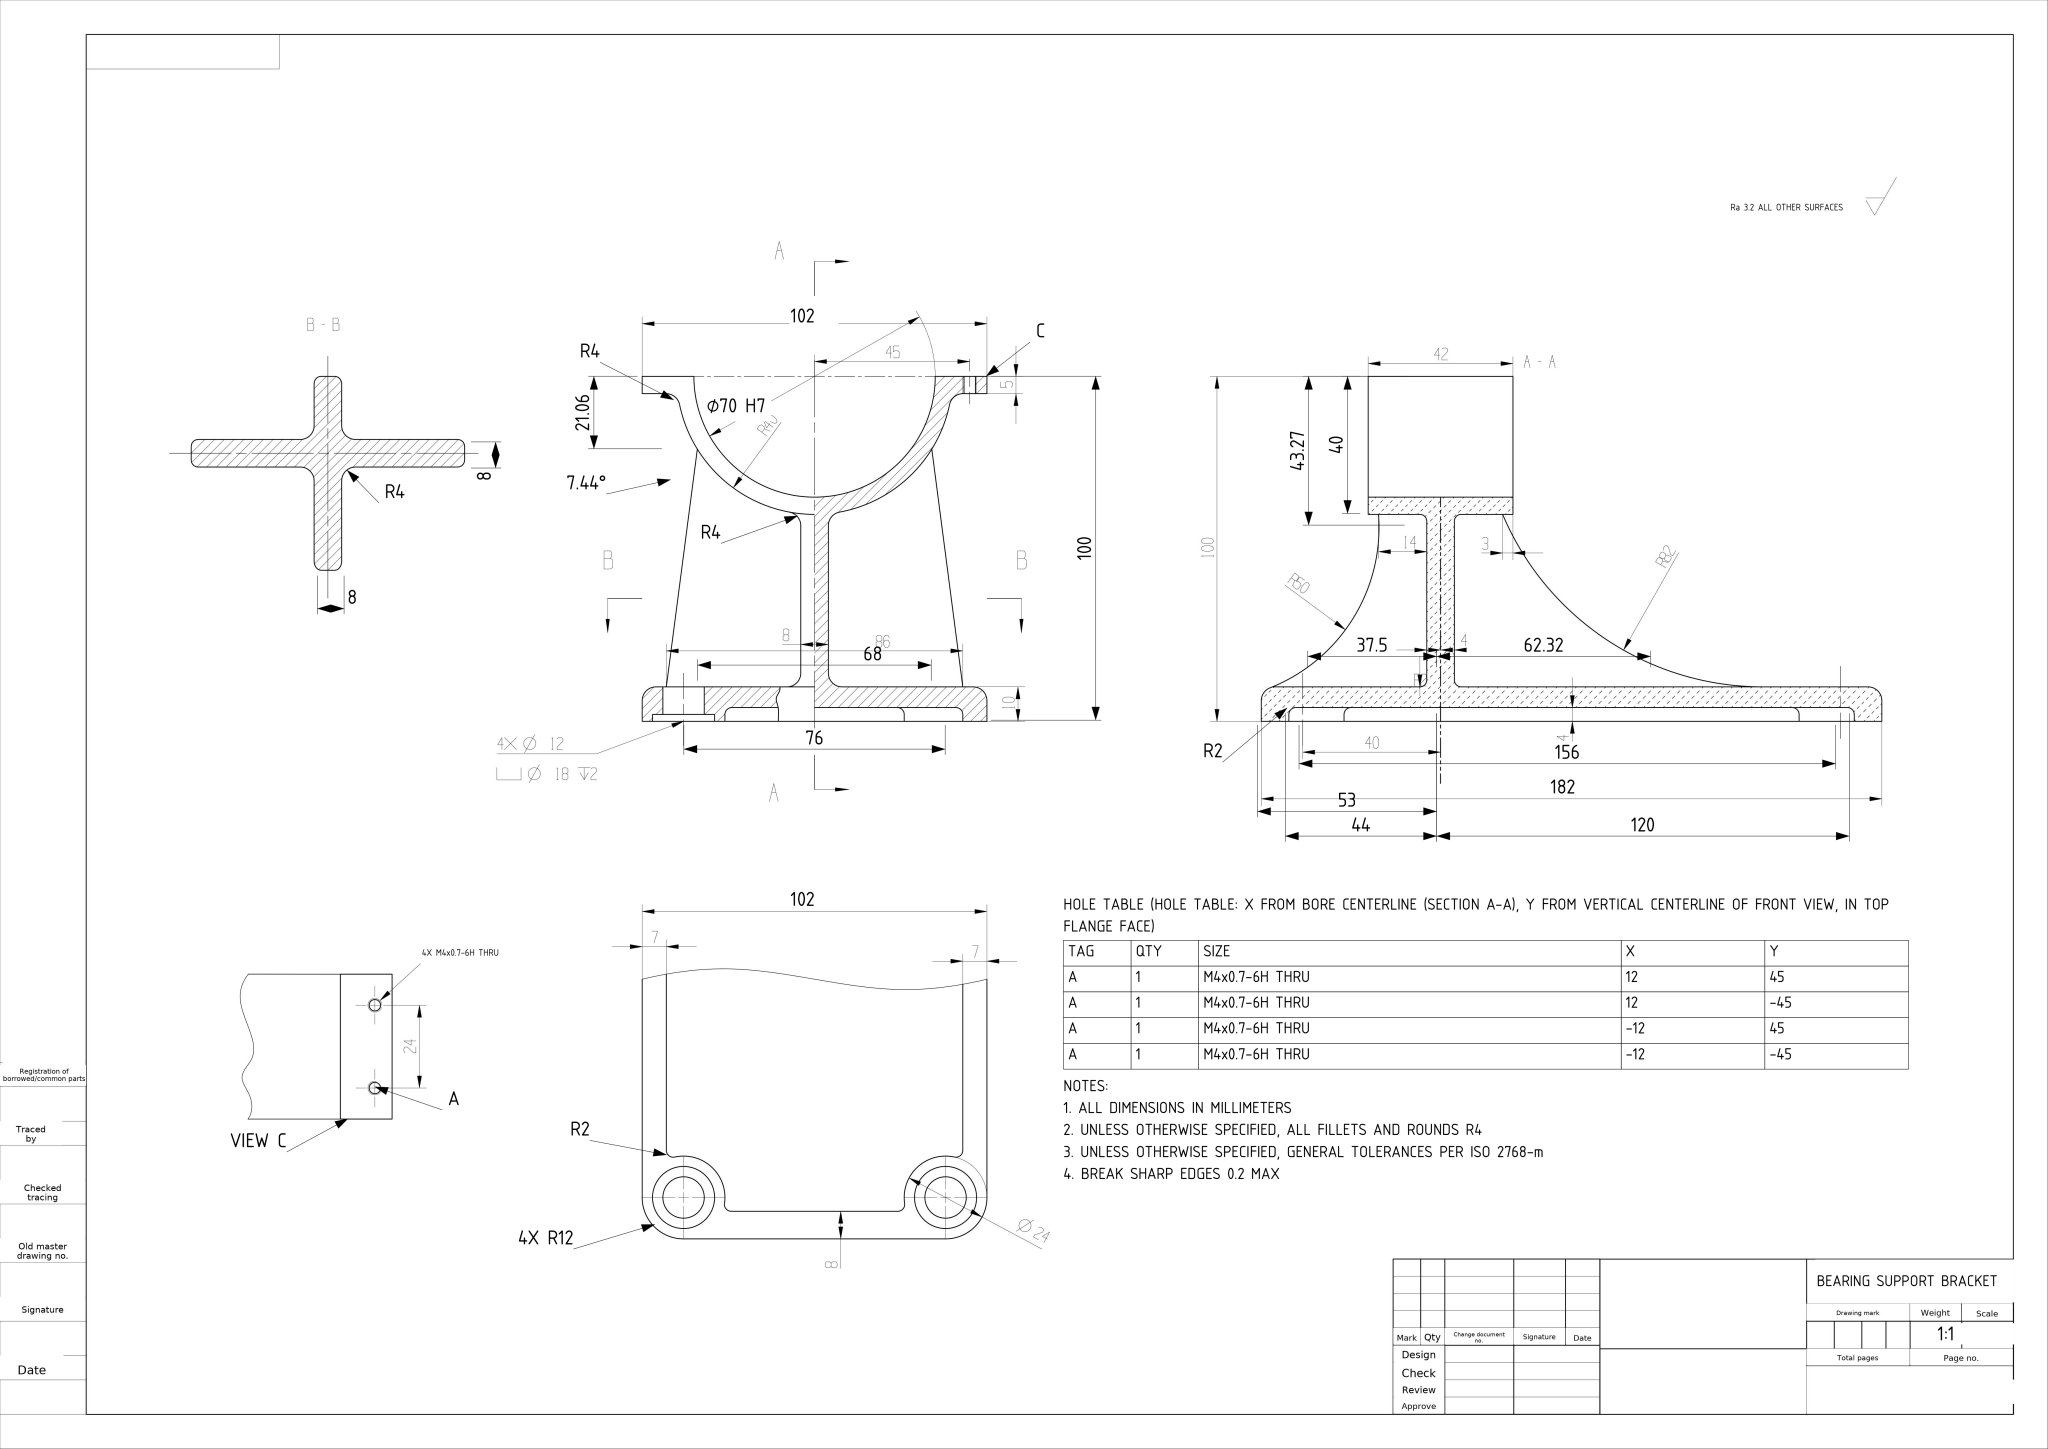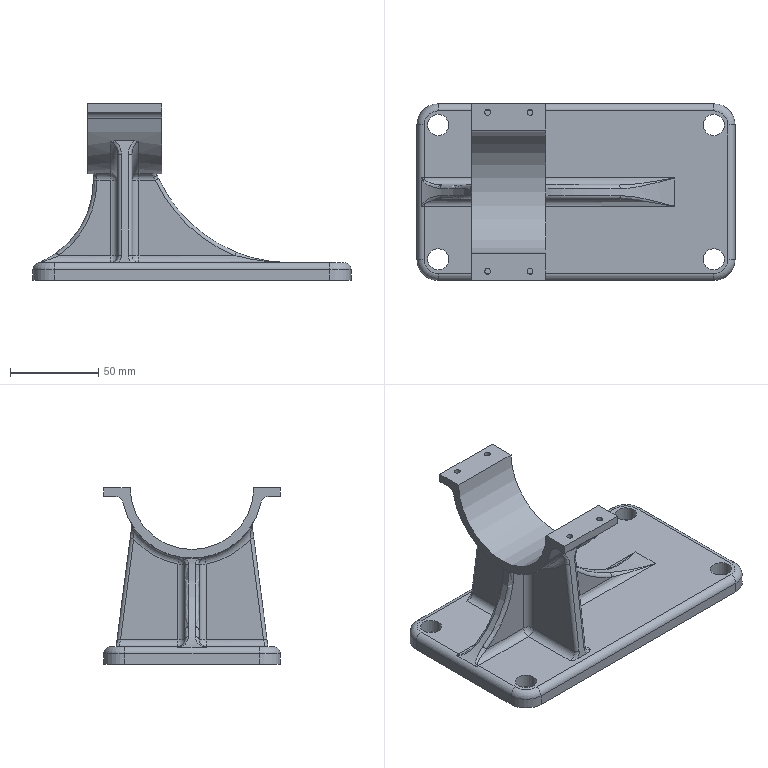Part | NX | mm | 1 solid | 155 faces | box 180 x 100 x 100 mm | volume 208195 mm3 | cylinder 62 | plane 37 | spline 22 | torus 18 | sphere 16 | commonest cylinder face diameters 8 x22 4 x16 24 x8 12 x4 18 x4 3.3 x4 70 x1 80 x1